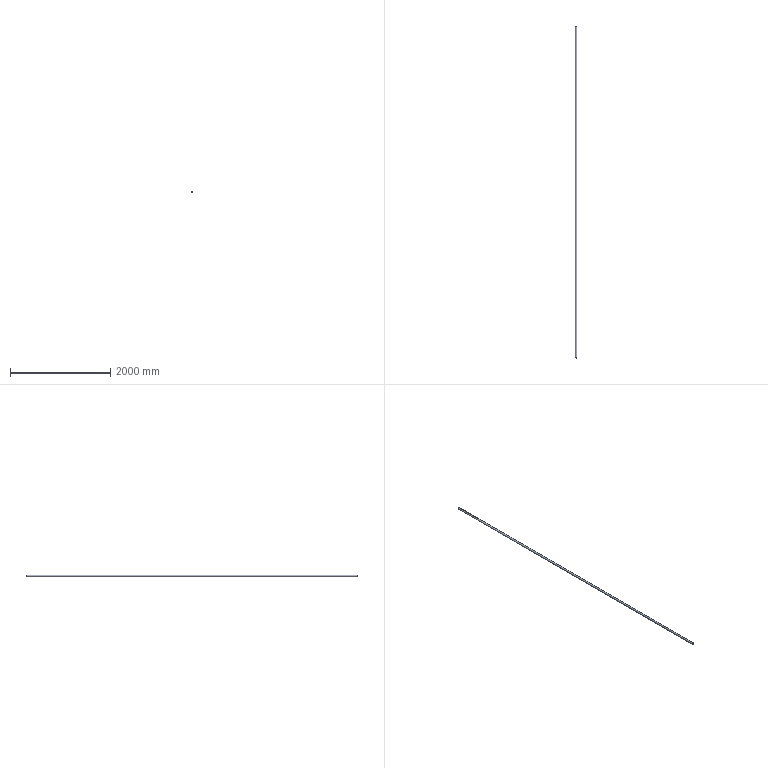Component | NX | 43_7 | 1 solid | 4 faces | volume 2223470 mm3 | cylinder 2 | plane 2 | commonest cylinder face diameters 34 x1 27 x1